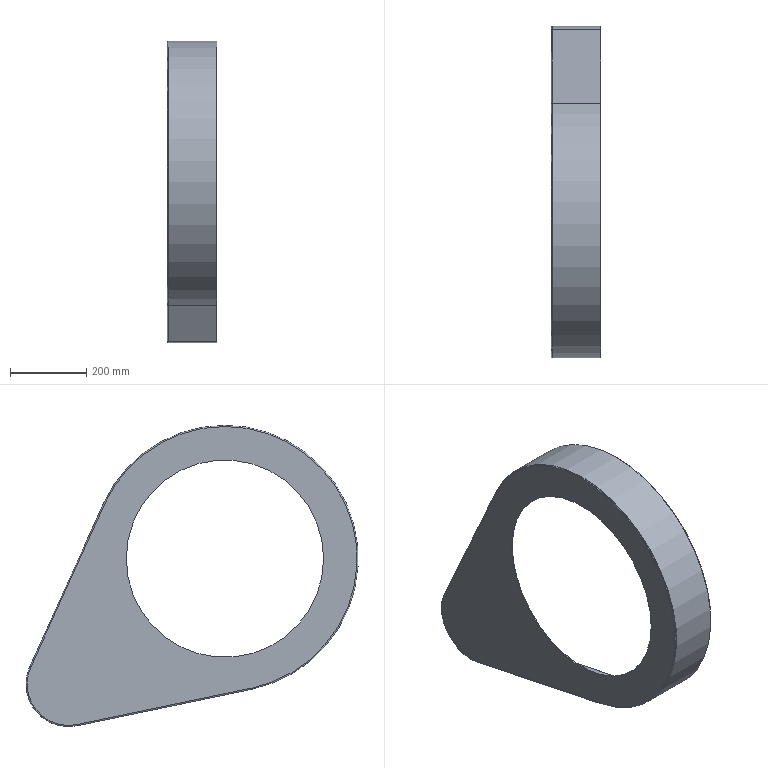Component | SolidWorks | PulleyGuard-1 | 1 solid | 25 faces | box 130 x 868.89 x 788.02 mm | volume 1195416 mm3 | cylinder 12 | plane 7 | torus 6 | commonest cylinder face diameters 516.003 x2 218.065 x2 222.065 x2 2 x2 6 x2 697.315 x1 693.315 x1
build123d program:
from build123d import *

# Parameters (mm, degrees)
BOSS_EXTRUDE1_DEPTH = 130
CUT_EXTRUDE1_DEPTH  = 128
HOLE1_D             = 516.003
FILLET1_R           = 1
FILLET2_R           = 3


with BuildPart() as part:
    # Sketch1 → Boss-Extrude1 (new body)
    with BuildSketch(Plane.XY.offset(130)):
        with BuildLine():
            Line((-71.54, -341.276), (386.298, -437.016))
            ThreePointArc((386.298, -437.016), (495.626, -397.821), (510.2, -282.598))
            Line((510.2, -282.598), (317.528, 143.618))
            ThreePointArc((317.528, 143.618), (-272.115, 218.198), (-71.54, -341.276))
        make_face()
    extrude(amount=-BOSS_EXTRUDE1_DEPTH)

    # Sketch2 → Cut-Extrude1 (cut)
    with BuildSketch(Plane.XY.offset(130)):
        with BuildLine():
            Line((-71.131, -339.318), (386.707, -435.058))
            ThreePointArc((386.707, -435.058), (494.066, -396.57), (508.378, -283.421))
            Line((508.378, -283.421), (315.706, 142.794))
            ThreePointArc((315.706, 142.794), (-270.555, 216.946), (-71.131, -339.318))
        make_face()
    extrude(amount=-CUT_EXTRUDE1_DEPTH, mode=Mode.SUBTRACT)

    # Hole1 (through all)
    with Locations(Plane.XY.offset(2)):
        with Locations((-0.1753, -0.0006894)):
            Hole(HOLE1_D / 2)

    # Fillet1
    fillet1_edges = [part.edges().sort_by_distance(p)[0] for p in [
        (-270.555, 216.946, 2),
        (412.042, -70.314, 2),
        (494.066, -396.57, 2),
        (157.788, -387.188, 2),
    ]]
    fillet(fillet1_edges, radius=FILLET1_R)

    # Fillet2
    fillet2_edges = [part.edges().sort_by_distance(p)[0] for p in [
        (495.626, -397.821, 0),
        (413.864, -69.49, 0),
        (-272.115, 218.198, 0),
        (157.379, -389.146, 0),
    ]]
    fillet(fillet2_edges, radius=FILLET2_R)


solid = part.part

# Placed as in the assembly
solid = solid.moved(Location((-913.659, 1336.004, 1014.811), (90, 90, 0)))
STEP:
#1=COLOUR_RGB('',0.7922,0.8196,0.9333);
#2=FILL_AREA_STYLE_COLOUR('',#1);
#3=FILL_AREA_STYLE('',(#2));
#4=SURFACE_STYLE_FILL_AREA(#3);
#5=SURFACE_SIDE_STYLE('',(#4));
#6=SURFACE_STYLE_USAGE(.BOTH.,#5);
#7=PRESENTATION_STYLE_ASSIGNMENT((#6));
#8=CARTESIAN_POINT('',(-35.971,72.955,27.027));
#9=VERTEX_POINT('',#8);
#10=CARTESIAN_POINT('',(-35.971,67.831,22.863));
#11=VERTEX_POINT('',#10);
#12=CARTESIAN_POINT('',(-35.971,68.702,27.027));
#13=DIRECTION('',(-1.,0.,0.));
#14=DIRECTION('',(0.,1.,0.));
#15=AXIS2_PLACEMENT_3D('',#12,#13,#14);
#16=CIRCLE('',#15,4.253);
#17=EDGE_CURVE('',#9,#11,#16,.T.);
#18=ORIENTED_EDGE('',*,*,#17,.F.);
#19=CARTESIAN_POINT('',(-35.853,73.073,27.027));
#20=VERTEX_POINT('',#19);
#21=CARTESIAN_POINT('',(-35.853,72.955,27.027));
#22=DIRECTION('',(0.,0.,-1.));
#23=DIRECTION('',(-1.,0.,0.));
#24=AXIS2_PLACEMENT_3D('',#21,#22,#23);
#25=CIRCLE('',#24,0.1181);
#26=EDGE_CURVE('',#9,#20,#25,.T.);
#27=ORIENTED_EDGE('',*,*,#26,.T.);
#28=CARTESIAN_POINT('',(-35.853,67.807,22.748));
#29=VERTEX_POINT('',#28);
#30=CARTESIAN_POINT('',(-35.853,68.702,27.027));
#31=DIRECTION('',(1.,0.,0.));
#32=DIRECTION('',(0.,1.,0.));
#33=AXIS2_PLACEMENT_3D('',#30,#31,#32);
#34=CIRCLE('',#33,4.371);
#35=EDGE_CURVE('',#29,#20,#34,.T.);
#36=ORIENTED_EDGE('',*,*,#35,.F.);
#37=CARTESIAN_POINT('',(-35.853,67.831,22.863));
#38=DIRECTION('',(0.,0.9788,-0.2047));
#39=DIRECTION('',(0.,0.2047,0.9788));
#40=AXIS2_PLACEMENT_3D('',#37,#38,#39);
#41=CIRCLE('',#40,0.1181);
#42=EDGE_CURVE('',#29,#11,#41,.T.);
#43=ORIENTED_EDGE('',*,*,#42,.T.);
#44=EDGE_LOOP('',(#18,#27,#36,#43));
#45=FACE_OUTER_BOUND('',#44,.T.);
#46=CARTESIAN_POINT('',(-35.853,68.702,27.027));
#47=DIRECTION('',(1.,0.,0.));
#48=DIRECTION('',(0.,1.,0.));
#49=AXIS2_PLACEMENT_3D('',#46,#47,#48);
#50=TOROIDAL_SURFACE('',#49,4.253,0.1181);
#51=ADVANCED_FACE('',(#45),#50,.T.);
#52=CARTESIAN_POINT('',(-35.892,72.955,27.027));
#53=VERTEX_POINT('',#52);
#54=CARTESIAN_POINT('',(-35.892,72.578,28.779));
#55=VERTEX_POINT('',#54);
#56=CARTESIAN_POINT('',(-35.892,68.702,27.027));
#57=DIRECTION('',(1.,0.,0.));
#58=DIRECTION('',(0.,1.,0.));
#59=AXIS2_PLACEMENT_3D('',#56,#57,#58);
#60=CIRCLE('',#59,4.253);
#61=EDGE_CURVE('',#53,#55,#60,.T.);
#62=ORIENTED_EDGE('',*,*,#61,.F.);
#63=CARTESIAN_POINT('',(-35.853,72.995,27.027));
#64=VERTEX_POINT('',#63);
#65=CARTESIAN_POINT('',(-35.853,72.955,27.027));
#66=DIRECTION('',(0.,0.,-1.));
#67=DIRECTION('',(-1.,0.,0.));
#68=AXIS2_PLACEMENT_3D('',#65,#66,#67);
#69=CIRCLE('',#68,0.03937);
#70=EDGE_CURVE('',#53,#64,#69,.T.);
#71=ORIENTED_EDGE('',*,*,#70,.T.);
#72=CARTESIAN_POINT('',(-35.853,72.613,28.795));
#73=VERTEX_POINT('',#72);
#74=CARTESIAN_POINT('',(-35.853,68.702,27.027));
#75=DIRECTION('',(-1.,0.,0.));
#76=DIRECTION('',(0.,1.,-0.));
#77=AXIS2_PLACEMENT_3D('',#74,#75,#76);
#78=CIRCLE('',#77,4.293);
#79=EDGE_CURVE('',#73,#64,#78,.T.);
#80=ORIENTED_EDGE('',*,*,#79,.F.);
#81=CARTESIAN_POINT('',(-35.853,72.578,28.779));
#82=DIRECTION('',(0.,0.4119,-0.9112));
#83=DIRECTION('',(0.,0.9112,0.4119));
#84=AXIS2_PLACEMENT_3D('',#81,#82,#83);
#85=CIRCLE('',#84,0.03937);
#86=EDGE_CURVE('',#55,#73,#85,.T.);
#87=ORIENTED_EDGE('',*,*,#86,.F.);
#88=EDGE_LOOP('',(#62,#71,#80,#87));
#89=FACE_OUTER_BOUND('',#88,.T.);
#90=CARTESIAN_POINT('',(-35.853,68.702,27.027));
#91=DIRECTION('',(1.,0.,0.));
#92=DIRECTION('',(0.,1.,0.));
#93=AXIS2_PLACEMENT_3D('',#90,#91,#92);
#94=TOROIDAL_SURFACE('',#93,4.253,0.03937);
#95=ADVANCED_FACE('',(#89),#94,.F.);
#96=CARTESIAN_POINT('',(-35.971,42.434,39.953));
#97=VERTEX_POINT('',#96);
#98=CARTESIAN_POINT('',(-35.971,62.749,39.953));
#99=VERTEX_POINT('',#98);
#100=CARTESIAN_POINT('',(-35.971,52.592,39.953));
#101=DIRECTION('',(1.,0.,0.));
#102=DIRECTION('',(0.,1.,0.));
#103=AXIS2_PLACEMENT_3D('',#100,#101,#102);
#104=CIRCLE('',#103,10.158);
#105=EDGE_CURVE('',#97,#99,#104,.T.);
#106=ORIENTED_EDGE('',*,*,#105,.F.);
#107=CARTESIAN_POINT('',(-35.892,42.434,39.953));
#108=VERTEX_POINT('',#107);
#109=CARTESIAN_POINT('',(-35.892,42.434,39.953));
#110=DIRECTION('',(1.,0.,0.));
#111=VECTOR('',#110,39.37);
#112=LINE('',#109,#111);
#113=EDGE_CURVE('',#97,#108,#112,.T.);
#114=ORIENTED_EDGE('',*,*,#113,.T.);
#115=CARTESIAN_POINT('',(-35.892,62.749,39.953));
#116=VERTEX_POINT('',#115);
#117=CARTESIAN_POINT('',(-35.892,52.592,39.953));
#118=DIRECTION('',(1.,0.,0.));
#119=DIRECTION('',(0.,1.,0.));
#120=AXIS2_PLACEMENT_3D('',#117,#118,#119);
#121=CIRCLE('',#120,10.158);
#122=EDGE_CURVE('',#108,#116,#121,.T.);
#123=ORIENTED_EDGE('',*,*,#122,.T.);
#124=CARTESIAN_POINT('',(-35.892,62.749,39.953));
#125=DIRECTION('',(1.,0.,0.));
#126=VECTOR('',#125,39.37);
#127=LINE('',#124,#126);
#128=EDGE_CURVE('',#99,#116,#127,.T.);
#129=ORIENTED_EDGE('',*,*,#128,.F.);
#130=EDGE_LOOP('',(#106,#114,#123,#129));
#131=FACE_OUTER_BOUND('',#130,.T.);
#132=CARTESIAN_POINT('',(-35.892,52.592,39.953));
#133=DIRECTION('',(1.,0.,0.));
#134=DIRECTION('',(0.,1.,0.));
#135=AXIS2_PLACEMENT_3D('',#132,#133,#134);
#136=CYLINDRICAL_SURFACE('',#135,10.158);
#137=ADVANCED_FACE('',(#131),#136,.F.);
#138=ORIENTED_EDGE('',*,*,#79,.T.);
#139=CARTESIAN_POINT('',(-30.853,72.995,27.027));
#140=VERTEX_POINT('',#139);
#141=CARTESIAN_POINT('',(-35.892,72.995,27.027));
#142=DIRECTION('',(1.,0.,0.));
#143=VECTOR('',#142,39.37);
#144=LINE('',#141,#143);
#145=EDGE_CURVE('',#64,#140,#144,.T.);
#146=ORIENTED_EDGE('',*,*,#145,.T.);
#147=CARTESIAN_POINT('',(-30.853,72.613,28.795));
#148=VERTEX_POINT('',#147);
#149=CARTESIAN_POINT('',(-30.853,68.702,27.027));
#150=DIRECTION('',(1.,0.,0.));
#151=DIRECTION('',(0.,1.,0.));
#152=AXIS2_PLACEMENT_3D('',#149,#150,#151);
#153=CIRCLE('',#152,4.293);
#154=EDGE_CURVE('',#140,#148,#153,.T.);
#155=ORIENTED_EDGE('',*,*,#154,.T.);
#156=CARTESIAN_POINT('',(-35.892,72.613,28.795));
#157=DIRECTION('',(1.,0.,0.));
#158=VECTOR('',#157,39.37);
#159=LINE('',#156,#158);
#160=EDGE_CURVE('',#73,#148,#159,.T.);
#161=ORIENTED_EDGE('',*,*,#160,.F.);
#162=EDGE_LOOP('',(#138,#146,#155,#161));
#163=FACE_OUTER_BOUND('',#162,.T.);
#164=CARTESIAN_POINT('',(-35.892,68.702,27.027));
#165=DIRECTION('',(1.,0.,0.));
#166=DIRECTION('',(0.,1.,0.));
#167=AXIS2_PLACEMENT_3D('',#164,#165,#166);
#168=CYLINDRICAL_SURFACE('',#167,4.293);
#169=ADVANCED_FACE('',(#163),#168,.F.);
#170=ORIENTED_EDGE('',*,*,#35,.T.);
#171=CARTESIAN_POINT('',(-30.853,73.073,27.027));
#172=VERTEX_POINT('',#171);
#173=CARTESIAN_POINT('',(-35.971,73.073,27.027));
#174=DIRECTION('',(1.,0.,0.));
#175=VECTOR('',#174,39.37);
#176=LINE('',#173,#175);
#177=EDGE_CURVE('',#20,#172,#176,.T.);
#178=ORIENTED_EDGE('',*,*,#177,.T.);
#179=CARTESIAN_POINT('',(-30.853,67.807,22.748));
#180=VERTEX_POINT('',#179);
#181=CARTESIAN_POINT('',(-30.853,68.702,27.027));
#182=DIRECTION('',(1.,0.,0.));
#183=DIRECTION('',(0.,1.,0.));
#184=AXIS2_PLACEMENT_3D('',#181,#182,#183);
#185=CIRCLE('',#184,4.371);
#186=EDGE_CURVE('',#180,#172,#185,.T.);
#187=ORIENTED_EDGE('',*,*,#186,.F.);
#188=CARTESIAN_POINT('',(-35.971,67.807,22.748));
#189=DIRECTION('',(1.,0.,0.));
#190=VECTOR('',#189,39.37);
#191=LINE('',#188,#190);
#192=EDGE_CURVE('',#29,#180,#191,.T.);
#193=ORIENTED_EDGE('',*,*,#192,.F.);
#194=EDGE_LOOP('',(#170,#178,#187,#193));
#195=FACE_OUTER_BOUND('',#194,.T.);
#196=CARTESIAN_POINT('',(-35.971,68.702,27.027));
#197=DIRECTION('',(1.,0.,0.));
#198=DIRECTION('',(0.,1.,0.));
#199=AXIS2_PLACEMENT_3D('',#196,#197,#198);
#200=CYLINDRICAL_SURFACE('',#199,4.371);
#201=ADVANCED_FACE('',(#195),#200,.T.);
#202=CARTESIAN_POINT('',(-35.853,65.1,45.607));
#203=VERTEX_POINT('',#202);
#204=CARTESIAN_POINT('',(-30.853,65.1,45.607));
#205=VERTEX_POINT('',#204);
#206=CARTESIAN_POINT('',(-35.971,65.1,45.607));
#207=DIRECTION('',(1.,0.,0.));
#208=VECTOR('',#207,39.37);
#209=LINE('',#206,#208);
#210=EDGE_CURVE('',#203,#205,#209,.T.);
#211=ORIENTED_EDGE('',*,*,#210,.F.);
#212=CARTESIAN_POINT('',(-35.853,49.782,26.517));
#213=VERTEX_POINT('',#212);
#214=CARTESIAN_POINT('',(-35.853,52.592,39.953));
#215=DIRECTION('',(1.,0.,0.));
#216=DIRECTION('',(0.,1.,0.));
#217=AXIS2_PLACEMENT_3D('',#214,#215,#216);
#218=CIRCLE('',#217,13.727);
#219=EDGE_CURVE('',#203,#213,#218,.T.);
#220=ORIENTED_EDGE('',*,*,#219,.T.);
#221=CARTESIAN_POINT('',(-30.853,49.782,26.517));
#222=VERTEX_POINT('',#221);
#223=CARTESIAN_POINT('',(-35.971,49.782,26.517));
#224=DIRECTION('',(1.,0.,0.));
#225=VECTOR('',#224,39.37);
#226=LINE('',#223,#225);
#227=EDGE_CURVE('',#213,#222,#226,.T.);
#228=ORIENTED_EDGE('',*,*,#227,.T.);
#229=CARTESIAN_POINT('',(-30.853,52.592,39.953));
#230=DIRECTION('',(1.,0.,0.));
#231=DIRECTION('',(0.,1.,0.));
#232=AXIS2_PLACEMENT_3D('',#229,#230,#231);
#233=CIRCLE('',#232,13.727);
#234=EDGE_CURVE('',#205,#222,#233,.T.);
#235=ORIENTED_EDGE('',*,*,#234,.F.);
#236=EDGE_LOOP('',(#211,#220,#228,#235));
#237=FACE_OUTER_BOUND('',#236,.T.);
#238=CARTESIAN_POINT('',(-35.971,52.592,39.953));
#239=DIRECTION('',(1.,0.,0.));
#240=DIRECTION('',(0.,1.,0.));
#241=AXIS2_PLACEMENT_3D('',#238,#239,#240);
#242=CYLINDRICAL_SURFACE('',#241,13.727);
#243=ADVANCED_FACE('',(#237),#242,.T.);
#244=CARTESIAN_POINT('',(-35.853,72.685,28.827));
#245=VERTEX_POINT('',#244);
#246=CARTESIAN_POINT('',(-30.853,72.685,28.827));
#247=VERTEX_POINT('',#246);
#248=CARTESIAN_POINT('',(-35.971,72.685,28.827));
#249=DIRECTION('',(1.,0.,0.));
#250=VECTOR('',#249,39.37);
#251=LINE('',#248,#250);
#252=EDGE_CURVE('',#245,#247,#251,.T.);
#253=ORIENTED_EDGE('',*,*,#252,.F.);
#254=CARTESIAN_POINT('',(-35.853,65.1,45.607));
#255=DIRECTION('',(0.,-0.4119,0.9112));
#256=VECTOR('',#255,39.37);
#257=LINE('',#254,#256);
#258=EDGE_CURVE('',#245,#203,#257,.T.);
#259=ORIENTED_EDGE('',*,*,#258,.T.);
#260=ORIENTED_EDGE('',*,*,#210,.T.);
#261=CARTESIAN_POINT('',(-30.853,72.685,28.827));
#262=DIRECTION('',(0.,-0.4119,0.9112));
#263=VECTOR('',#262,39.37);
#264=LINE('',#261,#263);
#265=EDGE_CURVE('',#247,#205,#264,.T.);
#266=ORIENTED_EDGE('',*,*,#265,.F.);
#267=EDGE_LOOP('',(#253,#259,#260,#266));
#268=FACE_OUTER_BOUND('',#267,.T.);
#269=CARTESIAN_POINT('',(-35.971,72.685,28.827));
#270=DIRECTION('',(0.,0.9112,0.4119));
#271=DIRECTION('',(0.,-0.4119,0.9112));
#272=AXIS2_PLACEMENT_3D('',#269,#270,#271);
#273=PLANE('',#272);
#274=ADVANCED_FACE('',(#268),#273,.T.);
#275=ORIENTED_EDGE('',*,*,#177,.F.);
#276=CARTESIAN_POINT('',(-35.853,68.702,27.027));
#277=DIRECTION('',(1.,0.,0.));
#278=DIRECTION('',(0.,1.,0.));
#279=AXIS2_PLACEMENT_3D('',#276,#277,#278);
#280=CIRCLE('',#279,4.371);
#281=EDGE_CURVE('',#20,#245,#280,.T.);
#282=ORIENTED_EDGE('',*,*,#281,.T.);
#283=ORIENTED_EDGE('',*,*,#252,.T.);
#284=CARTESIAN_POINT('',(-30.853,68.702,27.027));
#285=DIRECTION('',(1.,0.,0.));
#286=DIRECTION('',(0.,1.,0.));
#287=AXIS2_PLACEMENT_3D('',#284,#285,#286);
#288=CIRCLE('',#287,4.371);
#289=EDGE_CURVE('',#172,#247,#288,.T.);
#290=ORIENTED_EDGE('',*,*,#289,.F.);
#291=EDGE_LOOP('',(#275,#282,#283,#290));
#292=FACE_OUTER_BOUND('',#291,.T.);
#293=CARTESIAN_POINT('',(-35.971,68.702,27.027));
#294=DIRECTION('',(1.,0.,0.));
#295=DIRECTION('',(0.,1.,0.));
#296=AXIS2_PLACEMENT_3D('',#293,#294,#295);
#297=CYLINDRICAL_SURFACE('',#296,4.371);
#298=ADVANCED_FACE('',(#292),#297,.T.);
#299=ORIENTED_EDGE('',*,*,#227,.F.);
#300=CARTESIAN_POINT('',(-35.853,67.807,22.748));
#301=DIRECTION('',(0.,0.9788,-0.2047));
#302=VECTOR('',#301,39.37);
#303=LINE('',#300,#302);
#304=EDGE_CURVE('',#213,#29,#303,.T.);
#305=ORIENTED_EDGE('',*,*,#304,.T.);
#306=ORIENTED_EDGE('',*,*,#192,.T.);
#307=CARTESIAN_POINT('',(-30.853,49.782,26.517));
#308=DIRECTION('',(0.,0.9788,-0.2047));
#309=VECTOR('',#308,39.37);
#310=LINE('',#307,#309);
#311=EDGE_CURVE('',#222,#180,#310,.T.);
#312=ORIENTED_EDGE('',*,*,#311,.F.);
#313=EDGE_LOOP('',(#299,#305,#306,#312));
#314=FACE_OUTER_BOUND('',#313,.T.);
#315=CARTESIAN_POINT('',(-35.971,49.782,26.517));
#316=DIRECTION('',(0.,-0.2047,-0.9788));
#317=DIRECTION('',(0.,0.9788,-0.2047));
#318=AXIS2_PLACEMENT_3D('',#315,#316,#317);
#319=PLANE('',#318);
#320=ADVANCED_FACE('',(#314),#319,.T.);
#321=CARTESIAN_POINT('',(-35.971,49.806,26.633));
#322=VERTEX_POINT('',#321);
#323=CARTESIAN_POINT('',(-35.971,64.992,45.559));
#324=VERTEX_POINT('',#323);
#325=CARTESIAN_POINT('',(-35.971,52.592,39.953));
#326=DIRECTION('',(-1.,0.,0.));
#327=DIRECTION('',(0.,1.,0.));
#328=AXIS2_PLACEMENT_3D('',#325,#326,#327);
#329=CIRCLE('',#328,13.609);
#330=EDGE_CURVE('',#322,#324,#329,.T.);
#331=ORIENTED_EDGE('',*,*,#330,.T.);
#332=CARTESIAN_POINT('',(-35.971,72.578,28.779));
#333=VERTEX_POINT('',#332);
#334=CARTESIAN_POINT('',(-35.971,72.578,28.779));
#335=DIRECTION('',(0.,0.4119,-0.9112));
#336=VECTOR('',#335,39.37);
#337=LINE('',#334,#336);
#338=EDGE_CURVE('',#324,#333,#337,.T.);
#339=ORIENTED_EDGE('',*,*,#338,.T.);
#340=CARTESIAN_POINT('',(-35.971,68.702,27.027));
#341=DIRECTION('',(-1.,0.,0.));
#342=DIRECTION('',(0.,1.,-0.));
#343=AXIS2_PLACEMENT_3D('',#340,#341,#342);
#344=CIRCLE('',#343,4.253);
#345=EDGE_CURVE('',#333,#9,#344,.T.);
#346=ORIENTED_EDGE('',*,*,#345,.T.);
#347=ORIENTED_EDGE('',*,*,#17,.T.);
#348=CARTESIAN_POINT('',(-35.971,49.806,26.633));
#349=DIRECTION('',(0.,-0.9788,0.2047));
#350=VECTOR('',#349,39.37);
#351=LINE('',#348,#350);
#352=EDGE_CURVE('',#11,#322,#351,.T.);
#353=ORIENTED_EDGE('',*,*,#352,.T.);
#354=EDGE_LOOP('',(#331,#339,#346,#347,#353));
#355=FACE_OUTER_BOUND('',#354,.T.);
#356=CARTESIAN_POINT('',(-35.971,52.592,39.953));
#357=DIRECTION('',(1.,0.,0.));
#358=DIRECTION('',(0.,1.,0.));
#359=AXIS2_PLACEMENT_3D('',#356,#357,#358);
#360=CIRCLE('',#359,10.158);
#361=EDGE_CURVE('',#99,#97,#360,.T.);
#362=ORIENTED_EDGE('',*,*,#361,.T.);
#363=ORIENTED_EDGE('',*,*,#105,.T.);
#364=EDGE_LOOP('',(#362,#363));
#365=FACE_BOUND('',#364,.T.);
#366=CARTESIAN_POINT('',(-35.971,52.592,39.953));
#367=DIRECTION('',(1.,0.,0.));
#368=DIRECTION('',(0.,1.,0.));
#369=AXIS2_PLACEMENT_3D('',#366,#367,#368);
#370=PLANE('',#369);
#371=ADVANCED_FACE('',(#355,#365),#370,.F.);
#372=CARTESIAN_POINT('',(-30.853,65.028,45.575));
#373=VERTEX_POINT('',#372);
#374=CARTESIAN_POINT('',(-30.853,49.798,26.594));
#375=VERTEX_POINT('',#374);
#376=CARTESIAN_POINT('',(-30.853,52.592,39.953));
#377=DIRECTION('',(1.,0.,0.));
#378=DIRECTION('',(0.,1.,0.));
#379=AXIS2_PLACEMENT_3D('',#376,#377,#378);
#380=CIRCLE('',#379,13.648);
#381=EDGE_CURVE('',#373,#375,#380,.T.);
#382=ORIENTED_EDGE('',*,*,#381,.F.);
#383=CARTESIAN_POINT('',(-30.853,72.613,28.795));
#384=DIRECTION('',(0.,-0.4119,0.9112));
#385=VECTOR('',#384,39.37);
#386=LINE('',#383,#385);
#387=EDGE_CURVE('',#148,#373,#386,.T.);
#388=ORIENTED_EDGE('',*,*,#387,.F.);
#389=ORIENTED_EDGE('',*,*,#154,.F.);
#390=CARTESIAN_POINT('',(-30.853,67.823,22.825));
#391=VERTEX_POINT('',#390);
#392=CARTESIAN_POINT('',(-30.853,68.702,27.027));
#393=DIRECTION('',(1.,0.,0.));
#394=DIRECTION('',(0.,1.,0.));
#395=AXIS2_PLACEMENT_3D('',#392,#393,#394);
#396=CIRCLE('',#395,4.293);
#397=EDGE_CURVE('',#391,#140,#396,.T.);
#398=ORIENTED_EDGE('',*,*,#397,.F.);
#399=CARTESIAN_POINT('',(-30.853,49.798,26.594));
#400=DIRECTION('',(0.,0.9788,-0.2047));
#401=VECTOR('',#400,39.37);
#402=LINE('',#399,#401);
#403=EDGE_CURVE('',#375,#391,#402,.T.);
#404=ORIENTED_EDGE('',*,*,#403,.F.);
#405=EDGE_LOOP('',(#382,#388,#389,#398,#404));
#406=FACE_BOUND('',#405,.T.);
#407=ORIENTED_EDGE('',*,*,#234,.T.);
#408=ORIENTED_EDGE('',*,*,#311,.T.);
#409=ORIENTED_EDGE('',*,*,#186,.T.);
#410=ORIENTED_EDGE('',*,*,#289,.T.);
#411=ORIENTED_EDGE('',*,*,#265,.T.);
#412=EDGE_LOOP('',(#407,#408,#409,#410,#411));
#413=FACE_OUTER_BOUND('',#412,.T.);
#414=CARTESIAN_POINT('',(-30.853,52.592,39.953));
#415=DIRECTION('',(1.,0.,0.));
#416=DIRECTION('',(0.,1.,0.));
#417=AXIS2_PLACEMENT_3D('',#414,#415,#416);
#418=PLANE('',#417);
#419=ADVANCED_FACE('',(#406,#413),#418,.T.);
#420=CARTESIAN_POINT('',(-35.853,49.798,26.594));
#421=VERTEX_POINT('',#420);
#422=CARTESIAN_POINT('',(-35.892,49.798,26.594));
#423=DIRECTION('',(1.,0.,0.));
#424=VECTOR('',#423,39.37);
#425=LINE('',#422,#424);
#426=EDGE_CURVE('',#421,#375,#425,.T.);
#427=ORIENTED_EDGE('',*,*,#426,.F.);
#428=CARTESIAN_POINT('',(-35.853,65.028,45.575));
#429=VERTEX_POINT('',#428);
#430=CARTESIAN_POINT('',(-35.853,52.592,39.953));
#431=DIRECTION('',(-1.,0.,0.));
#432=DIRECTION('',(0.,1.,0.));
#433=AXIS2_PLACEMENT_3D('',#430,#431,#432);
#434=CIRCLE('',#433,13.648);
#435=EDGE_CURVE('',#421,#429,#434,.T.);
#436=ORIENTED_EDGE('',*,*,#435,.T.);
#437=CARTESIAN_POINT('',(-35.892,65.028,45.575));
#438=DIRECTION('',(1.,0.,0.));
#439=VECTOR('',#438,39.37);
#440=LINE('',#437,#439);
#441=EDGE_CURVE('',#429,#373,#440,.T.);
#442=ORIENTED_EDGE('',*,*,#441,.T.);
#443=ORIENTED_EDGE('',*,*,#381,.T.);
#444=EDGE_LOOP('',(#427,#436,#442,#443));
#445=FACE_OUTER_BOUND('',#444,.T.);
#446=CARTESIAN_POINT('',(-35.892,52.592,39.953));
#447=DIRECTION('',(1.,0.,0.));
#448=DIRECTION('',(0.,1.,0.));
#449=AXIS2_PLACEMENT_3D('',#446,#447,#448);
#450=CYLINDRICAL_SURFACE('',#449,13.648);
#451=ADVANCED_FACE('',(#445),#450,.F.);
#452=ORIENTED_EDGE('',*,*,#441,.F.);
#453=CARTESIAN_POINT('',(-35.853,72.613,28.795));
#454=DIRECTION('',(0.,0.4119,-0.9112));
#455=VECTOR('',#454,39.37);
#456=LINE('',#453,#455);
#457=EDGE_CURVE('',#429,#73,#456,.T.);
#458=ORIENTED_EDGE('',*,*,#457,.T.);
#459=ORIENTED_EDGE('',*,*,#160,.T.);
#460=ORIENTED_EDGE('',*,*,#387,.T.);
#461=EDGE_LOOP('',(#452,#458,#459,#460));
#462=FACE_OUTER_BOUND('',#461,.T.);
#463=CARTESIAN_POINT('',(-35.892,72.613,28.795));
#464=DIRECTION('',(0.,0.9112,0.4119));
#465=DIRECTION('',(0.,-0.4119,0.9112));
#466=AXIS2_PLACEMENT_3D('',#463,#464,#465);
#467=PLANE('',#466);
#468=ADVANCED_FACE('',(#462),#467,.F.);
#469=ORIENTED_EDGE('',*,*,#145,.F.);
#470=CARTESIAN_POINT('',(-35.853,67.823,22.825));
#471=VERTEX_POINT('',#470);
#472=CARTESIAN_POINT('',(-35.853,68.702,27.027));
#473=DIRECTION('',(-1.,0.,0.));
#474=DIRECTION('',(0.,1.,0.));
#475=AXIS2_PLACEMENT_3D('',#472,#473,#474);
#476=CIRCLE('',#475,4.293);
#477=EDGE_CURVE('',#64,#471,#476,.T.);
#478=ORIENTED_EDGE('',*,*,#477,.T.);
#479=CARTESIAN_POINT('',(-35.892,67.823,22.825));
#480=DIRECTION('',(1.,0.,0.));
#481=VECTOR('',#480,39.37);
#482=LINE('',#479,#481);
#483=EDGE_CURVE('',#471,#391,#482,.T.);
#484=ORIENTED_EDGE('',*,*,#483,.T.);
#485=ORIENTED_EDGE('',*,*,#397,.T.);
#486=EDGE_LOOP('',(#469,#478,#484,#485));
#487=FACE_OUTER_BOUND('',#486,.T.);
#488=CARTESIAN_POINT('',(-35.892,68.702,27.027));
#489=DIRECTION('',(1.,0.,0.));
#490=DIRECTION('',(0.,1.,0.));
#491=AXIS2_PLACEMENT_3D('',#488,#489,#490);
#492=CYLINDRICAL_SURFACE('',#491,4.293);
#493=ADVANCED_FACE('',(#487),#492,.F.);
#494=ORIENTED_EDGE('',*,*,#483,.F.);
#495=CARTESIAN_POINT('',(-35.853,49.798,26.594));
#496=DIRECTION('',(0.,-0.9788,0.2047));
#497=VECTOR('',#496,39.37);
#498=LINE('',#495,#497);
#499=EDGE_CURVE('',#471,#421,#498,.T.);
#500=ORIENTED_EDGE('',*,*,#499,.T.);
#501=ORIENTED_EDGE('',*,*,#426,.T.);
#502=ORIENTED_EDGE('',*,*,#403,.T.);
#503=EDGE_LOOP('',(#494,#500,#501,#502));
#504=FACE_OUTER_BOUND('',#503,.T.);
#505=CARTESIAN_POINT('',(-35.892,49.798,26.594));
#506=DIRECTION('',(0.,-0.2047,-0.9788));
#507=DIRECTION('',(0.,0.9788,-0.2047));
#508=AXIS2_PLACEMENT_3D('',#505,#506,#507);
#509=PLANE('',#508);
#510=ADVANCED_FACE('',(#504),#509,.F.);
#511=CARTESIAN_POINT('',(-35.892,64.992,45.559));
#512=VERTEX_POINT('',#511);
#513=CARTESIAN_POINT('',(-35.892,64.992,45.559));
#514=DIRECTION('',(0.,-0.4119,0.9112));
#515=VECTOR('',#514,39.37);
#516=LINE('',#513,#515);
#517=EDGE_CURVE('',#55,#512,#516,.T.);
#518=ORIENTED_EDGE('',*,*,#517,.T.);
#519=CARTESIAN_POINT('',(-35.892,49.806,26.633));
#520=VERTEX_POINT('',#519);
#521=CARTESIAN_POINT('',(-35.892,52.592,39.953));
#522=DIRECTION('',(1.,0.,0.));
#523=DIRECTION('',(0.,1.,0.));
#524=AXIS2_PLACEMENT_3D('',#521,#522,#523);
#525=CIRCLE('',#524,13.609);
#526=EDGE_CURVE('',#512,#520,#525,.T.);
#527=ORIENTED_EDGE('',*,*,#526,.T.);
#528=CARTESIAN_POINT('',(-35.892,67.831,22.863));
#529=VERTEX_POINT('',#528);
#530=CARTESIAN_POINT('',(-35.892,49.806,26.633));
#531=DIRECTION('',(0.,0.9788,-0.2047));
#532=VECTOR('',#531,39.37);
#533=LINE('',#530,#532);
#534=EDGE_CURVE('',#520,#529,#533,.T.);
#535=ORIENTED_EDGE('',*,*,#534,.T.);
#536=CARTESIAN_POINT('',(-35.892,68.702,27.027));
#537=DIRECTION('',(1.,0.,0.));
#538=DIRECTION('',(0.,1.,0.));
#539=AXIS2_PLACEMENT_3D('',#536,#537,#538);
#540=CIRCLE('',#539,4.253);
#541=EDGE_CURVE('',#529,#53,#540,.T.);
#542=ORIENTED_EDGE('',*,*,#541,.T.);
#543=ORIENTED_EDGE('',*,*,#61,.T.);
#544=EDGE_LOOP('',(#518,#527,#535,#542,#543));
#545=FACE_OUTER_BOUND('',#544,.T.);
#546=CARTESIAN_POINT('',(-35.892,52.592,39.953));
#547=DIRECTION('',(1.,0.,0.));
#548=DIRECTION('',(0.,1.,0.));
#549=AXIS2_PLACEMENT_3D('',#546,#547,#548);
#550=CIRCLE('',#549,10.158);
#551=EDGE_CURVE('',#116,#108,#550,.T.);
#552=ORIENTED_EDGE('',*,*,#551,.F.);
#553=ORIENTED_EDGE('',*,*,#122,.F.);
#554=EDGE_LOOP('',(#552,#553));
#555=FACE_BOUND('',#554,.T.);
#556=CARTESIAN_POINT('',(-35.892,52.592,39.953));
#557=DIRECTION('',(1.,0.,0.));
#558=DIRECTION('',(0.,1.,0.));
#559=AXIS2_PLACEMENT_3D('',#556,#557,#558);
#560=PLANE('',#559);
#561=ADVANCED_FACE('',(#545,#555),#560,.T.);
#562=ORIENTED_EDGE('',*,*,#113,.F.);
#563=ORIENTED_EDGE('',*,*,#361,.F.);
#564=ORIENTED_EDGE('',*,*,#128,.T.);
#565=ORIENTED_EDGE('',*,*,#551,.T.);
#566=EDGE_LOOP('',(#562,#563,#564,#565));
#567=FACE_OUTER_BOUND('',#566,.T.);
#568=CARTESIAN_POINT('',(-35.892,52.592,39.953));
#569=DIRECTION('',(1.,0.,0.));
#570=DIRECTION('',(0.,1.,0.));
#571=AXIS2_PLACEMENT_3D('',#568,#569,#570);
#572=CYLINDRICAL_SURFACE('',#571,10.158);
#573=ADVANCED_FACE('',(#567),#572,.F.);
#574=ORIENTED_EDGE('',*,*,#70,.F.);
#575=ORIENTED_EDGE('',*,*,#541,.F.);
#576=CARTESIAN_POINT('',(-35.853,67.831,22.863));
#577=DIRECTION('',(0.,0.9788,-0.2047));
#578=DIRECTION('',(0.,0.2047,0.9788));
#579=AXIS2_PLACEMENT_3D('',#576,#577,#578);
#580=CIRCLE('',#579,0.03937);
#581=EDGE_CURVE('',#471,#529,#580,.T.);
#582=ORIENTED_EDGE('',*,*,#581,.F.);
#583=ORIENTED_EDGE('',*,*,#477,.F.);
#584=EDGE_LOOP('',(#574,#575,#582,#583));
#585=FACE_OUTER_BOUND('',#584,.T.);
#586=CARTESIAN_POINT('',(-35.853,68.702,27.027));
#587=DIRECTION('',(1.,0.,0.));
#588=DIRECTION('',(0.,1.,0.));
#589=AXIS2_PLACEMENT_3D('',#586,#587,#588);
#590=TOROIDAL_SURFACE('',#589,4.253,0.03937);
#591=ADVANCED_FACE('',(#585),#590,.F.);
#592=ORIENTED_EDGE('',*,*,#86,.T.);
#593=ORIENTED_EDGE('',*,*,#457,.F.);
#594=CARTESIAN_POINT('',(-35.853,64.992,45.559));
#595=DIRECTION('',(0.,0.4119,-0.9112));
#596=DIRECTION('',(0.,0.9112,0.4119));
#597=AXIS2_PLACEMENT_3D('',#594,#595,#596);
#598=CIRCLE('',#597,0.03937);
#599=EDGE_CURVE('',#512,#429,#598,.T.);
#600=ORIENTED_EDGE('',*,*,#599,.F.);
#601=ORIENTED_EDGE('',*,*,#517,.F.);
#602=EDGE_LOOP('',(#592,#593,#600,#601));
#603=FACE_OUTER_BOUND('',#602,.T.);
#604=CARTESIAN_POINT('',(-35.853,64.992,45.559));
#605=DIRECTION('',(0.,-0.4119,0.9112));
#606=DIRECTION('',(0.,-0.9112,-0.4119));
#607=AXIS2_PLACEMENT_3D('',#604,#605,#606);
#608=CYLINDRICAL_SURFACE('',#607,0.03937);
#609=ADVANCED_FACE('',(#603),#608,.F.);
#610=ORIENTED_EDGE('',*,*,#581,.T.);
#611=ORIENTED_EDGE('',*,*,#534,.F.);
#612=CARTESIAN_POINT('',(-35.853,49.806,26.633));
#613=DIRECTION('',(0.,0.9788,-0.2047));
#614=DIRECTION('',(0.,0.2047,0.9788));
#615=AXIS2_PLACEMENT_3D('',#612,#613,#614);
#616=CIRCLE('',#615,0.03937);
#617=EDGE_CURVE('',#421,#520,#616,.T.);
#618=ORIENTED_EDGE('',*,*,#617,.F.);
#619=ORIENTED_EDGE('',*,*,#499,.F.);
#620=EDGE_LOOP('',(#610,#611,#618,#619));
#621=FACE_OUTER_BOUND('',#620,.T.);
#622=CARTESIAN_POINT('',(-35.853,49.806,26.633));
#623=DIRECTION('',(0.,0.9788,-0.2047));
#624=DIRECTION('',(0.,0.2047,0.9788));
#625=AXIS2_PLACEMENT_3D('',#622,#623,#624);
#626=CYLINDRICAL_SURFACE('',#625,0.03937);
#627=ADVANCED_FACE('',(#621),#626,.F.);
#628=ORIENTED_EDGE('',*,*,#599,.T.);
#629=ORIENTED_EDGE('',*,*,#435,.F.);
#630=ORIENTED_EDGE('',*,*,#617,.T.);
#631=ORIENTED_EDGE('',*,*,#526,.F.);
#632=EDGE_LOOP('',(#628,#629,#630,#631));
#633=FACE_OUTER_BOUND('',#632,.T.);
#634=CARTESIAN_POINT('',(-35.853,52.592,39.953));
#635=DIRECTION('',(1.,0.,0.));
#636=DIRECTION('',(0.,1.,0.));
#637=AXIS2_PLACEMENT_3D('',#634,#635,#636);
#638=TOROIDAL_SURFACE('',#637,13.609,0.03937);
#639=ADVANCED_FACE('',(#633),#638,.F.);
#640=CARTESIAN_POINT('',(-35.853,49.806,26.633));
#641=DIRECTION('',(0.,-0.9788,0.2047));
#642=DIRECTION('',(0.,-0.2047,-0.9788));
#643=AXIS2_PLACEMENT_3D('',#640,#641,#642);
#644=CIRCLE('',#643,0.1181);
#645=EDGE_CURVE('',#322,#213,#644,.T.);
#646=ORIENTED_EDGE('',*,*,#645,.F.);
#647=ORIENTED_EDGE('',*,*,#352,.F.);
#648=ORIENTED_EDGE('',*,*,#42,.F.);
#649=ORIENTED_EDGE('',*,*,#304,.F.);
#650=EDGE_LOOP('',(#646,#647,#648,#649));
#651=FACE_OUTER_BOUND('',#650,.T.);
#652=CARTESIAN_POINT('',(-35.853,49.806,26.633));
#653=DIRECTION('',(0.,-0.9788,0.2047));
#654=DIRECTION('',(0.,-0.2047,-0.9788));
#655=AXIS2_PLACEMENT_3D('',#652,#653,#654);
#656=CYLINDRICAL_SURFACE('',#655,0.1181);
#657=ADVANCED_FACE('',(#651),#656,.T.);
#658=ORIENTED_EDGE('',*,*,#26,.F.);
#659=ORIENTED_EDGE('',*,*,#345,.F.);
#660=CARTESIAN_POINT('',(-35.853,72.578,28.779));
#661=DIRECTION('',(0.,-0.4119,0.9112));
#662=DIRECTION('',(0.,-0.9112,-0.4119));
#663=AXIS2_PLACEMENT_3D('',#660,#661,#662);
#664=CIRCLE('',#663,0.1181);
#665=EDGE_CURVE('',#245,#333,#664,.T.);
#666=ORIENTED_EDGE('',*,*,#665,.F.);
#667=ORIENTED_EDGE('',*,*,#281,.F.);
#668=EDGE_LOOP('',(#658,#659,#666,#667));
#669=FACE_OUTER_BOUND('',#668,.T.);
#670=CARTESIAN_POINT('',(-35.853,68.702,27.027));
#671=DIRECTION('',(1.,0.,0.));
#672=DIRECTION('',(0.,1.,0.));
#673=AXIS2_PLACEMENT_3D('',#670,#671,#672);
#674=TOROIDAL_SURFACE('',#673,4.253,0.1181);
#675=ADVANCED_FACE('',(#669),#674,.T.);
#676=ORIENTED_EDGE('',*,*,#645,.T.);
#677=ORIENTED_EDGE('',*,*,#219,.F.);
#678=CARTESIAN_POINT('',(-35.853,64.992,45.559));
#679=DIRECTION('',(0.,0.4119,-0.9112));
#680=DIRECTION('',(0.,0.9112,0.4119));
#681=AXIS2_PLACEMENT_3D('',#678,#679,#680);
#682=CIRCLE('',#681,0.1181);
#683=EDGE_CURVE('',#324,#203,#682,.T.);
#684=ORIENTED_EDGE('',*,*,#683,.F.);
#685=ORIENTED_EDGE('',*,*,#330,.F.);
#686=EDGE_LOOP('',(#676,#677,#684,#685));
#687=FACE_OUTER_BOUND('',#686,.T.);
#688=CARTESIAN_POINT('',(-35.853,52.592,39.953));
#689=DIRECTION('',(1.,0.,0.));
#690=DIRECTION('',(0.,1.,0.));
#691=AXIS2_PLACEMENT_3D('',#688,#689,#690);
#692=TOROIDAL_SURFACE('',#691,13.609,0.1181);
#693=ADVANCED_FACE('',(#687),#692,.T.);
#694=ORIENTED_EDGE('',*,*,#665,.T.);
#695=ORIENTED_EDGE('',*,*,#338,.F.);
#696=ORIENTED_EDGE('',*,*,#683,.T.);
#697=ORIENTED_EDGE('',*,*,#258,.F.);
#698=EDGE_LOOP('',(#694,#695,#696,#697));
#699=FACE_OUTER_BOUND('',#698,.T.);
#700=CARTESIAN_POINT('',(-35.853,72.578,28.779));
#701=DIRECTION('',(0.,0.4119,-0.9112));
#702=DIRECTION('',(0.,0.9112,0.4119));
#703=AXIS2_PLACEMENT_3D('',#700,#701,#702);
#704=CYLINDRICAL_SURFACE('',#703,0.1181);
#705=ADVANCED_FACE('',(#699),#704,.T.);
#706=CLOSED_SHELL('',(#51,#95,#137,#169,#201,#243,#274,#298,#320,#371,#419,#451,#468,#493,#510,#561,#573,#591,#609,#627,#639,#657,#675,#693,#705));
#707=MANIFOLD_SOLID_BREP('',#706);
#708=STYLED_ITEM('',(#7),#707);
#709=PRESENTATION_LAYER_ASSIGNMENT('','',(#708));
#710=(LENGTH_UNIT()NAMED_UNIT(*)SI_UNIT($,.METRE.));
#711=LENGTH_MEASURE_WITH_UNIT(LENGTH_MEASURE(0.0254),#710);
#712=DIMENSIONAL_EXPONENTS(1.,0.,0.,0.,0.,0.,0.);
#713=(CONVERSION_BASED_UNIT('',#711)LENGTH_UNIT()NAMED_UNIT(#712));
#714=UNCERTAINTY_MEASURE_WITH_UNIT(LENGTH_MEASURE(0.00001),#713,'','');
#715=(NAMED_UNIT(*)PLANE_ANGLE_UNIT()SI_UNIT($,.RADIAN.));
#716=(NAMED_UNIT(*)SI_UNIT($,.STERADIAN.)SOLID_ANGLE_UNIT());
#717=(GEOMETRIC_REPRESENTATION_CONTEXT(3)GLOBAL_UNCERTAINTY_ASSIGNED_CONTEXT((#714))GLOBAL_UNIT_ASSIGNED_CONTEXT((#713,#715,#716))REPRESENTATION_CONTEXT('',''));
#718=MECHANICAL_DESIGN_GEOMETRIC_PRESENTATION_REPRESENTATION('',(#708),#717);
#719=CARTESIAN_POINT('',(0.,0.,0.));
#720=DIRECTION('',(0.,0.,1.));
#721=DIRECTION('',(1.,0.,0.));
#722=AXIS2_PLACEMENT_3D('',#719,#720,#721);
#723=(LENGTH_UNIT()NAMED_UNIT(*)SI_UNIT($,.METRE.));
#724=LENGTH_MEASURE_WITH_UNIT(LENGTH_MEASURE(0.0254),#723);
#725=DIMENSIONAL_EXPONENTS(1.,0.,0.,0.,0.,0.,0.);
#726=(CONVERSION_BASED_UNIT('',#724)LENGTH_UNIT()NAMED_UNIT(#725));
#727=UNCERTAINTY_MEASURE_WITH_UNIT(LENGTH_MEASURE(0.00001),#726,'','');
#728=(NAMED_UNIT(*)PLANE_ANGLE_UNIT()SI_UNIT($,.RADIAN.));
#729=(NAMED_UNIT(*)SI_UNIT($,.STERADIAN.)SOLID_ANGLE_UNIT());
#730=(GEOMETRIC_REPRESENTATION_CONTEXT(3)GLOBAL_UNCERTAINTY_ASSIGNED_CONTEXT((#727))GLOBAL_UNIT_ASSIGNED_CONTEXT((#726,#728,#729))REPRESENTATION_CONTEXT('',''));
#731=ADVANCED_BREP_SHAPE_REPRESENTATION('',(#707,#722),#730);